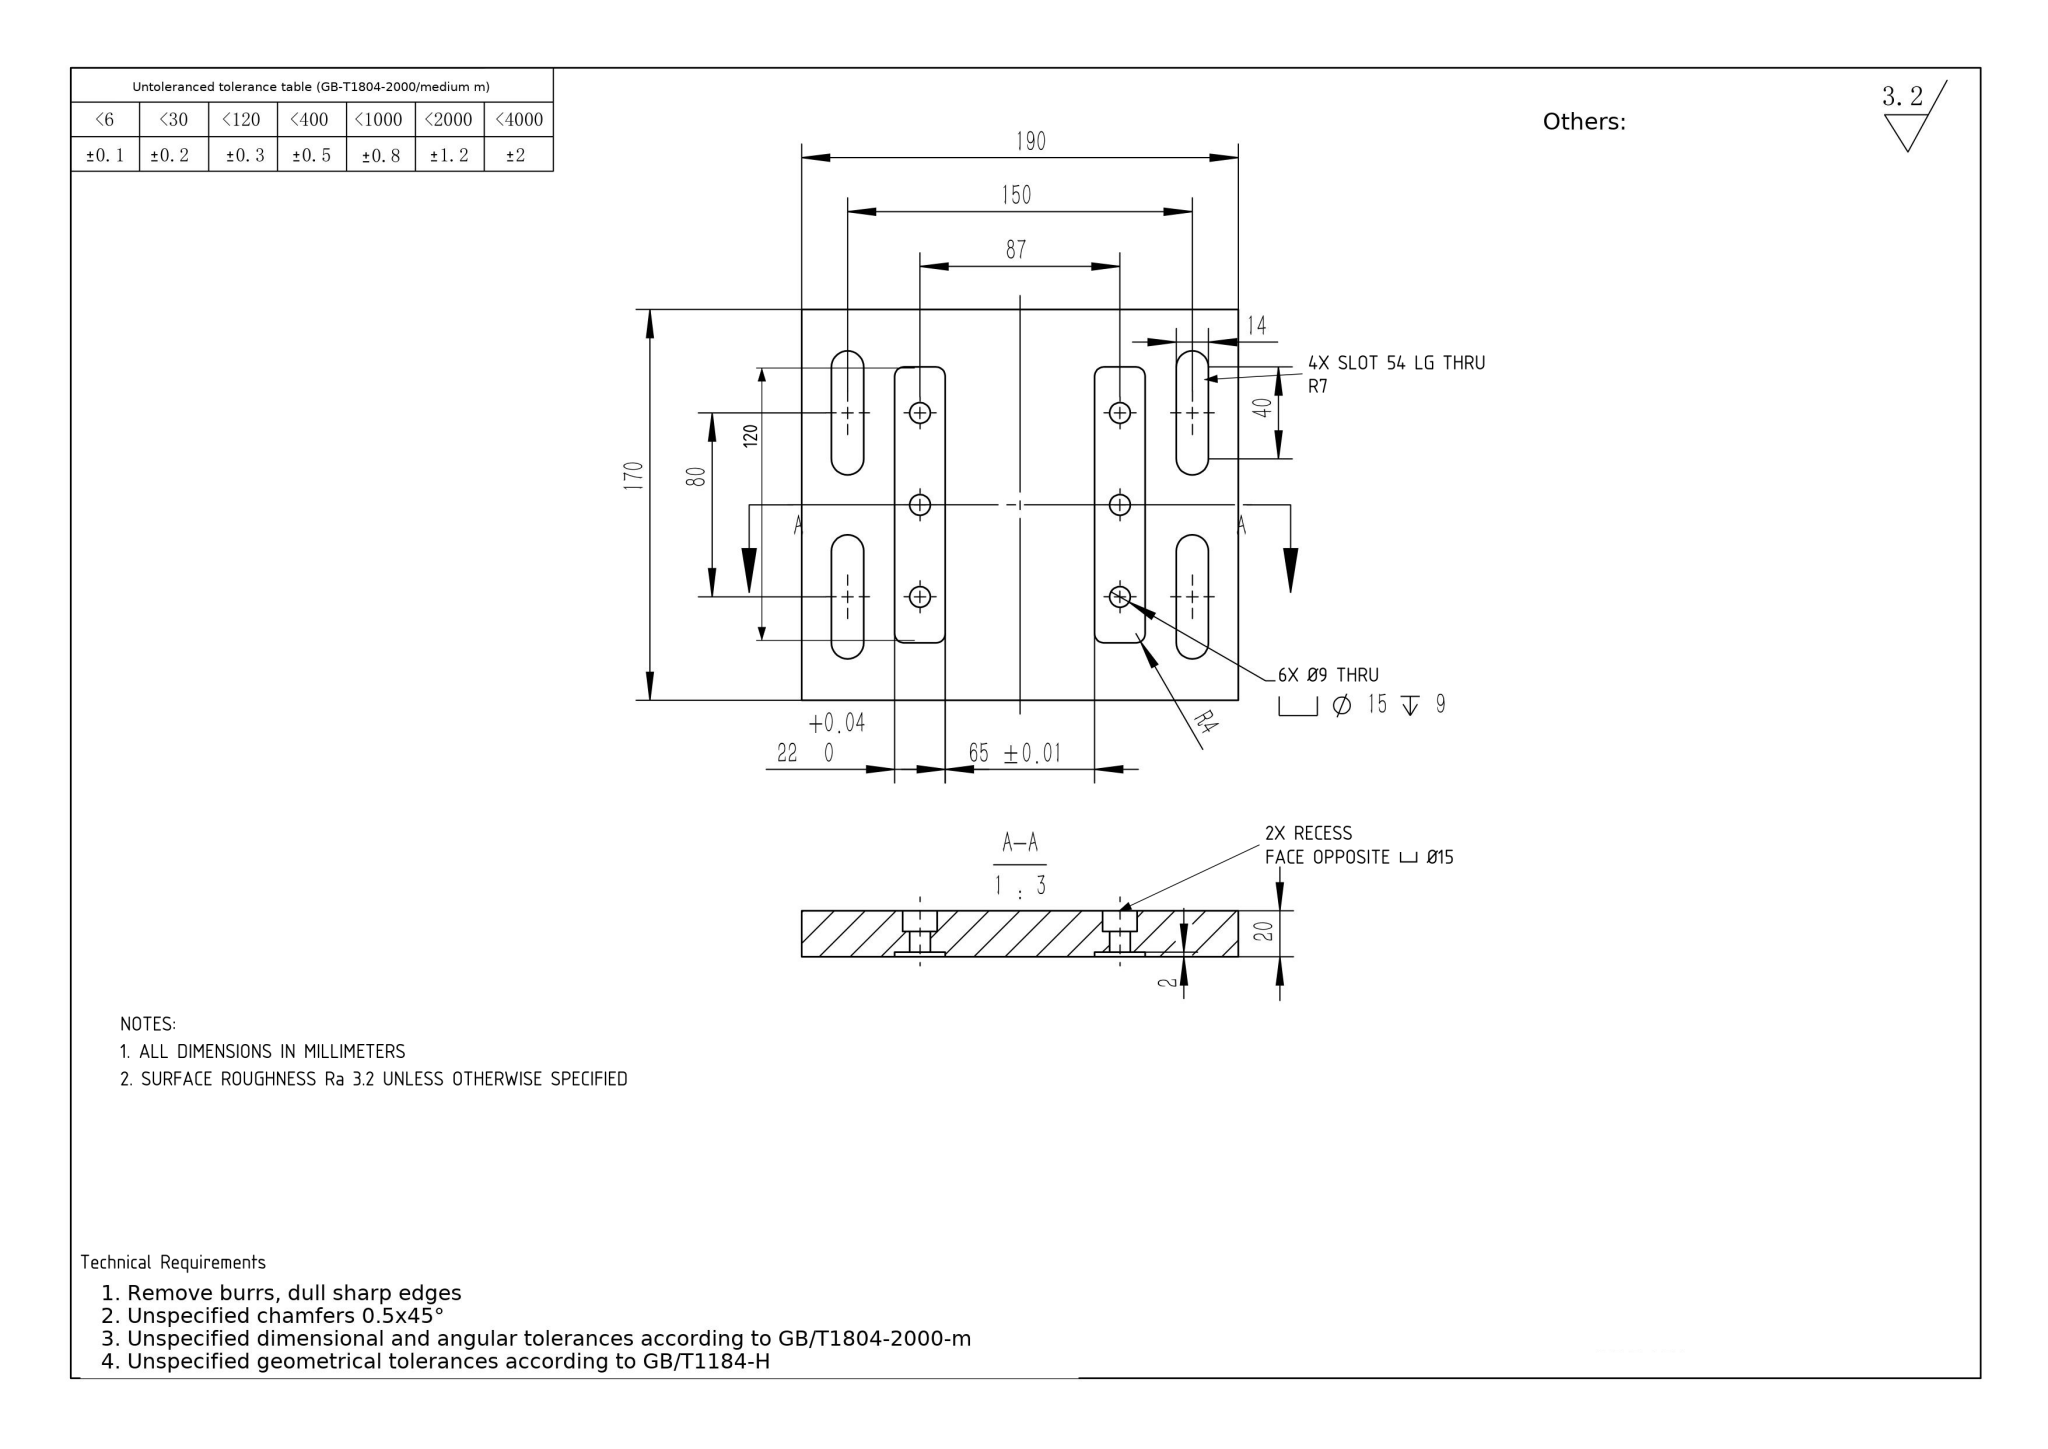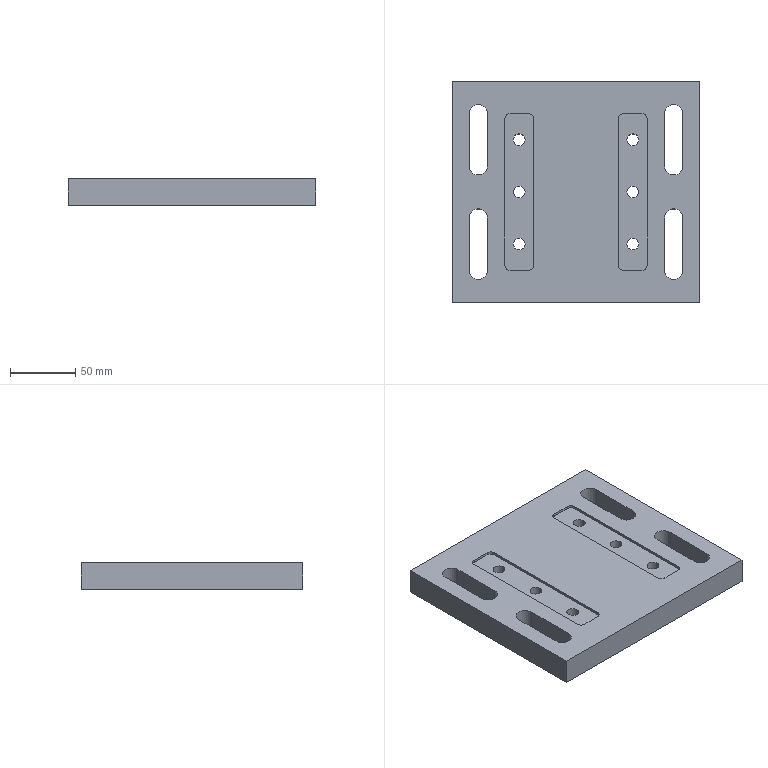Part | NX | mm | 1 solid | 70 faces | box 190 x 170 x 20 mm | volume 565402 mm3 | cylinder 40 | plane 30 | commonest cylinder face diameters 15 x12 9 x12 8 x8 14 x8